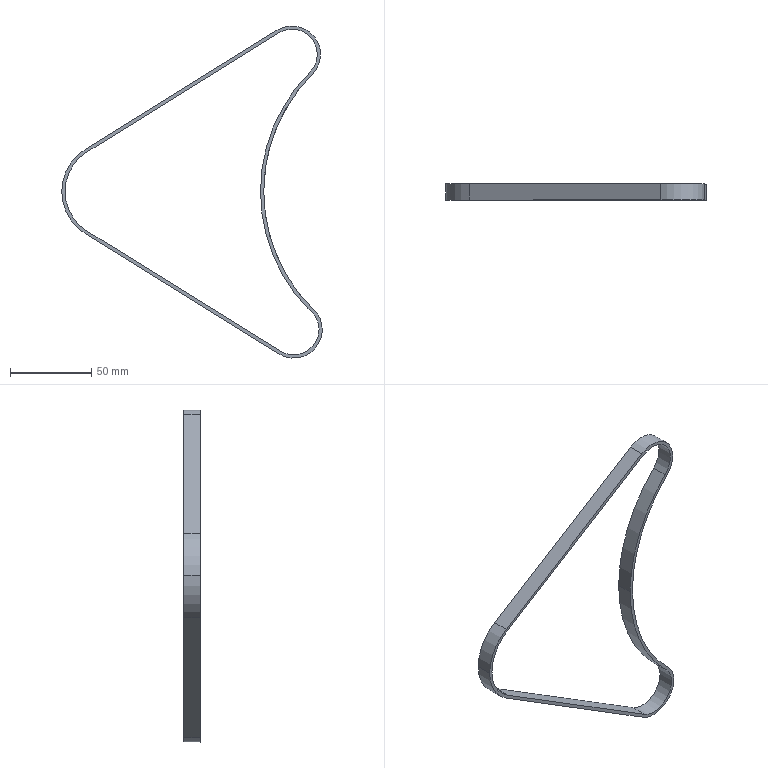Component | SolidWorks | Belt2-1 | 1 solid | 18 faces | box 159.92 x 10 x 203.95 mm | volume 11922 mm3 | cylinder 12 | plane 6 | commonest cylinder face diameters 207 x2 57 x2 203 x2 61 x2 31 x2 35 x2
STEP:
#1=COLOUR_RGB('',0.7922,0.8196,0.9333);
#2=FILL_AREA_STYLE_COLOUR('',#1);
#3=FILL_AREA_STYLE('',(#2));
#4=SURFACE_STYLE_FILL_AREA(#3);
#5=SURFACE_SIDE_STYLE('',(#4));
#6=SURFACE_STYLE_USAGE(.BOTH.,#5);
#7=PRESENTATION_STYLE_ASSIGNMENT((#6));
#8=CARTESIAN_POINT('',(0.02532,-2.067,3.386));
#9=VERTEX_POINT('',#8);
#10=CARTESIAN_POINT('',(-1.122,-2.067,6.22));
#11=VERTEX_POINT('',#10);
#12=CARTESIAN_POINT('',(2.953,-2.067,6.22));
#13=DIRECTION('',(0.,1.,0.));
#14=DIRECTION('',(1.,-0.,0.));
#15=AXIS2_PLACEMENT_3D('',#12,#13,#14);
#16=CIRCLE('',#15,4.075);
#17=EDGE_CURVE('',#9,#11,#16,.T.);
#18=ORIENTED_EDGE('',*,*,#17,.T.);
#19=CARTESIAN_POINT('',(-1.122,-1.673,6.22));
#20=VERTEX_POINT('',#19);
#21=CARTESIAN_POINT('',(-1.122,-2.067,6.22));
#22=DIRECTION('',(0.,1.,0.));
#23=VECTOR('',#22,39.37);
#24=LINE('',#21,#23);
#25=EDGE_CURVE('',#11,#20,#24,.T.);
#26=ORIENTED_EDGE('',*,*,#25,.T.);
#27=CARTESIAN_POINT('',(0.02532,-1.673,3.386));
#28=VERTEX_POINT('',#27);
#29=CARTESIAN_POINT('',(2.953,-1.673,6.22));
#30=DIRECTION('',(0.,1.,0.));
#31=DIRECTION('',(1.,-0.,0.));
#32=AXIS2_PLACEMENT_3D('',#29,#30,#31);
#33=CIRCLE('',#32,4.075);
#34=EDGE_CURVE('',#28,#20,#33,.T.);
#35=ORIENTED_EDGE('',*,*,#34,.F.);
#36=CARTESIAN_POINT('',(0.02532,-2.067,3.386));
#37=DIRECTION('',(0.,1.,0.));
#38=VECTOR('',#37,39.37);
#39=LINE('',#36,#38);
#40=EDGE_CURVE('',#9,#28,#39,.T.);
#41=ORIENTED_EDGE('',*,*,#40,.F.);
#42=EDGE_LOOP('',(#18,#26,#35,#41));
#43=FACE_OUTER_BOUND('',#42,.T.);
#44=CARTESIAN_POINT('',(2.953,-2.067,6.22));
#45=DIRECTION('',(0.,1.,0.));
#46=DIRECTION('',(-1.,0.,-0.));
#47=AXIS2_PLACEMENT_3D('',#44,#45,#46);
#48=CYLINDRICAL_SURFACE('',#47,4.075);
#49=ADVANCED_FACE('',(#43),#48,.T.);
#50=CARTESIAN_POINT('',(-5.316,-2.067,7.174));
#51=VERTEX_POINT('',#50);
#52=CARTESIAN_POINT('',(-5.846,-2.067,6.22));
#53=VERTEX_POINT('',#52);
#54=CARTESIAN_POINT('',(-4.724,-2.067,6.22));
#55=DIRECTION('',(-0.,-1.,-0.));
#56=DIRECTION('',(1.,-0.,0.));
#57=AXIS2_PLACEMENT_3D('',#54,#55,#56);
#58=CIRCLE('',#57,1.122);
#59=EDGE_CURVE('',#51,#53,#58,.T.);
#60=ORIENTED_EDGE('',*,*,#59,.T.);
#61=CARTESIAN_POINT('',(-5.846,-1.673,6.22));
#62=VERTEX_POINT('',#61);
#63=CARTESIAN_POINT('',(-5.846,-2.067,6.22));
#64=DIRECTION('',(0.,1.,0.));
#65=VECTOR('',#64,39.37);
#66=LINE('',#63,#65);
#67=EDGE_CURVE('',#53,#62,#66,.T.);
#68=ORIENTED_EDGE('',*,*,#67,.T.);
#69=CARTESIAN_POINT('',(-5.316,-1.673,7.174));
#70=VERTEX_POINT('',#69);
#71=CARTESIAN_POINT('',(-4.724,-1.673,6.22));
#72=DIRECTION('',(-0.,-1.,-0.));
#73=DIRECTION('',(1.,-0.,0.));
#74=AXIS2_PLACEMENT_3D('',#71,#72,#73);
#75=CIRCLE('',#74,1.122);
#76=EDGE_CURVE('',#70,#62,#75,.T.);
#77=ORIENTED_EDGE('',*,*,#76,.F.);
#78=CARTESIAN_POINT('',(-5.316,-2.067,7.174));
#79=DIRECTION('',(0.,1.,0.));
#80=VECTOR('',#79,39.37);
#81=LINE('',#78,#80);
#82=EDGE_CURVE('',#51,#70,#81,.T.);
#83=ORIENTED_EDGE('',*,*,#82,.F.);
#84=EDGE_LOOP('',(#60,#68,#77,#83));
#85=FACE_OUTER_BOUND('',#84,.T.);
#86=CARTESIAN_POINT('',(-4.724,-2.067,6.22));
#87=DIRECTION('',(0.,1.,0.));
#88=DIRECTION('',(-1.,0.,-0.));
#89=AXIS2_PLACEMENT_3D('',#86,#87,#88);
#90=CYLINDRICAL_SURFACE('',#89,1.122);
#91=ADVANCED_FACE('',(#85),#90,.F.);
#92=CARTESIAN_POINT('',(-1.043,-2.067,6.22));
#93=VERTEX_POINT('',#92);
#94=CARTESIAN_POINT('',(0.1271,-2.067,9.046));
#95=VERTEX_POINT('',#94);
#96=CARTESIAN_POINT('',(2.953,-2.067,6.22));
#97=DIRECTION('',(0.,1.,0.));
#98=DIRECTION('',(1.,-0.,0.));
#99=AXIS2_PLACEMENT_3D('',#96,#97,#98);
#100=CIRCLE('',#99,3.996);
#101=EDGE_CURVE('',#93,#95,#100,.T.);
#102=ORIENTED_EDGE('',*,*,#101,.F.);
#103=CARTESIAN_POINT('',(-1.043,-1.673,6.22));
#104=VERTEX_POINT('',#103);
#105=CARTESIAN_POINT('',(-1.043,-2.067,6.22));
#106=DIRECTION('',(0.,1.,0.));
#107=VECTOR('',#106,39.37);
#108=LINE('',#105,#107);
#109=EDGE_CURVE('',#93,#104,#108,.T.);
#110=ORIENTED_EDGE('',*,*,#109,.T.);
#111=CARTESIAN_POINT('',(0.1271,-1.673,9.046));
#112=VERTEX_POINT('',#111);
#113=CARTESIAN_POINT('',(-1.043,-1.673,6.22));
#114=CARTESIAN_POINT('',(-1.043,-1.673,6.482));
#115=CARTESIAN_POINT('',(-1.018,-1.673,6.744));
#116=CARTESIAN_POINT('',(-0.9155,-1.673,7.257));
#117=CARTESIAN_POINT('',(-0.8392,-1.673,7.508));
#118=CARTESIAN_POINT('',(-0.639,-1.673,7.991));
#119=CARTESIAN_POINT('',(-0.5152,-1.673,8.223));
#120=CARTESIAN_POINT('',(-0.2245,-1.673,8.658));
#121=CARTESIAN_POINT('',(-0.05783,-1.673,8.861));
#122=CARTESIAN_POINT('',(0.1271,-1.673,9.046));
#123=B_SPLINE_CURVE_WITH_KNOTS('',3,(#113,#114,#115,#116,#117,#118,#119,#120,#121,#122),.UNSPECIFIED.,.F.,.F.,(4,2,2,2,4),(0.4942,0.6206,0.7471,0.8735,1.),.UNSPECIFIED.);
#124=EDGE_CURVE('',#104,#112,#123,.T.);
#125=ORIENTED_EDGE('',*,*,#124,.T.);
#126=CARTESIAN_POINT('',(0.1271,-2.067,9.046));
#127=DIRECTION('',(0.,1.,0.));
#128=VECTOR('',#127,39.37);
#129=LINE('',#126,#128);
#130=EDGE_CURVE('',#95,#112,#129,.T.);
#131=ORIENTED_EDGE('',*,*,#130,.F.);
#132=EDGE_LOOP('',(#102,#110,#125,#131));
#133=FACE_OUTER_BOUND('',#132,.T.);
#134=CARTESIAN_POINT('',(2.953,-2.067,6.22));
#135=DIRECTION('',(0.,1.,0.));
#136=DIRECTION('',(-1.,0.,-0.));
#137=AXIS2_PLACEMENT_3D('',#134,#135,#136);
#138=CYLINDRICAL_SURFACE('',#137,3.996);
#139=ADVANCED_FACE('',(#133),#138,.F.);
#140=CARTESIAN_POINT('',(-5.925,-2.067,6.22));
#141=VERTEX_POINT('',#140);
#142=CARTESIAN_POINT('',(-5.358,-2.067,5.2));
#143=VERTEX_POINT('',#142);
#144=CARTESIAN_POINT('',(-4.724,-2.067,6.22));
#145=DIRECTION('',(-0.,-1.,-0.));
#146=DIRECTION('',(1.,-0.,0.));
#147=AXIS2_PLACEMENT_3D('',#144,#145,#146);
#148=CIRCLE('',#147,1.201);
#149=EDGE_CURVE('',#141,#143,#148,.T.);
#150=ORIENTED_EDGE('',*,*,#149,.F.);
#151=CARTESIAN_POINT('',(-5.925,-1.673,6.22));
#152=VERTEX_POINT('',#151);
#153=CARTESIAN_POINT('',(-5.925,-2.067,6.22));
#154=DIRECTION('',(0.,1.,0.));
#155=VECTOR('',#154,39.37);
#156=LINE('',#153,#155);
#157=EDGE_CURVE('',#141,#152,#156,.T.);
#158=ORIENTED_EDGE('',*,*,#157,.T.);
#159=CARTESIAN_POINT('',(-5.358,-1.673,5.2));
#160=VERTEX_POINT('',#159);
#161=CARTESIAN_POINT('',(-4.724,-1.673,6.22));
#162=DIRECTION('',(-0.,-1.,-0.));
#163=DIRECTION('',(1.,-0.,0.));
#164=AXIS2_PLACEMENT_3D('',#161,#162,#163);
#165=CIRCLE('',#164,1.201);
#166=EDGE_CURVE('',#152,#160,#165,.T.);
#167=ORIENTED_EDGE('',*,*,#166,.T.);
#168=CARTESIAN_POINT('',(-5.358,-2.067,5.2));
#169=DIRECTION('',(0.,1.,0.));
#170=VECTOR('',#169,39.37);
#171=LINE('',#168,#170);
#172=EDGE_CURVE('',#143,#160,#171,.T.);
#173=ORIENTED_EDGE('',*,*,#172,.F.);
#174=EDGE_LOOP('',(#150,#158,#167,#173));
#175=FACE_OUTER_BOUND('',#174,.T.);
#176=CARTESIAN_POINT('',(-4.724,-2.067,6.22));
#177=DIRECTION('',(0.,1.,0.));
#178=DIRECTION('',(-1.,0.,-0.));
#179=AXIS2_PLACEMENT_3D('',#176,#177,#178);
#180=CYLINDRICAL_SURFACE('',#179,1.201);
#181=ADVANCED_FACE('',(#175),#180,.T.);
#182=ORIENTED_EDGE('',*,*,#76,.T.);
#183=CARTESIAN_POINT('',(-5.316,-1.673,5.267));
#184=VERTEX_POINT('',#183);
#185=CARTESIAN_POINT('',(-4.724,-1.673,6.22));
#186=DIRECTION('',(-0.,-1.,-0.));
#187=DIRECTION('',(1.,-0.,0.));
#188=AXIS2_PLACEMENT_3D('',#185,#186,#187);
#189=CIRCLE('',#188,1.122);
#190=EDGE_CURVE('',#62,#184,#189,.T.);
#191=ORIENTED_EDGE('',*,*,#190,.T.);
#192=CARTESIAN_POINT('',(-0.6401,-1.673,2.363));
#193=VERTEX_POINT('',#192);
#194=CARTESIAN_POINT('',(-5.316,-1.673,5.267));
#195=DIRECTION('',(0.8495,0.,-0.5276));
#196=VECTOR('',#195,39.37);
#197=LINE('',#194,#196);
#198=EDGE_CURVE('',#184,#193,#197,.T.);
#199=ORIENTED_EDGE('',*,*,#198,.T.);
#200=CARTESIAN_POINT('',(-0.3181,-1.673,2.882));
#201=DIRECTION('',(-0.,-1.,-0.));
#202=DIRECTION('',(1.,-0.,0.));
#203=AXIS2_PLACEMENT_3D('',#200,#201,#202);
#204=CIRCLE('',#203,0.6102);
#205=EDGE_CURVE('',#193,#28,#204,.T.);
#206=ORIENTED_EDGE('',*,*,#205,.T.);
#207=ORIENTED_EDGE('',*,*,#34,.T.);
#208=CARTESIAN_POINT('',(0.07143,-1.673,9.102));
#209=VERTEX_POINT('',#208);
#210=CARTESIAN_POINT('',(2.953,-1.673,6.22));
#211=DIRECTION('',(0.,1.,0.));
#212=DIRECTION('',(1.,-0.,0.));
#213=AXIS2_PLACEMENT_3D('',#210,#211,#212);
#214=CIRCLE('',#213,4.075);
#215=EDGE_CURVE('',#20,#209,#214,.T.);
#216=ORIENTED_EDGE('',*,*,#215,.T.);
#217=CARTESIAN_POINT('',(-0.682,-1.673,10.052));
#218=VERTEX_POINT('',#217);
#219=CARTESIAN_POINT('',(-0.3601,-1.673,9.533));
#220=DIRECTION('',(-0.,-1.,-0.));
#221=DIRECTION('',(1.,-0.,0.));
#222=AXIS2_PLACEMENT_3D('',#219,#220,#221);
#223=CIRCLE('',#222,0.6102);
#224=EDGE_CURVE('',#209,#218,#223,.T.);
#225=ORIENTED_EDGE('',*,*,#224,.T.);
#226=CARTESIAN_POINT('',(-5.316,-1.673,7.174));
#227=DIRECTION('',(-0.8495,0.,-0.5276));
#228=VECTOR('',#227,39.37);
#229=LINE('',#226,#228);
#230=EDGE_CURVE('',#218,#70,#229,.T.);
#231=ORIENTED_EDGE('',*,*,#230,.T.);
#232=EDGE_LOOP('',(#182,#191,#199,#206,#207,#216,#225,#231));
#233=FACE_BOUND('',#232,.T.);
#234=CARTESIAN_POINT('',(0.2385,-1.673,3.288));
#235=VERTEX_POINT('',#234);
#236=CARTESIAN_POINT('',(0.07649,-1.673,3.446));
#237=VERTEX_POINT('',#236);
#238=CARTESIAN_POINT('',(0.2385,-1.673,3.288));
#239=CARTESIAN_POINT('',(0.2107,-1.673,3.313));
#240=CARTESIAN_POINT('',(0.156,-1.673,3.365));
#241=CARTESIAN_POINT('',(0.1027,-1.673,3.419));
#242=CARTESIAN_POINT('',(0.07649,-1.673,3.446));
#243=B_SPLINE_CURVE_WITH_KNOTS('',3,(#238,#239,#240,#241,#242),.UNSPECIFIED.,.F.,.F.,(4,1,4),(0.8688,0.8734,0.8779),.UNSPECIFIED.);
#244=EDGE_CURVE('',#235,#237,#243,.T.);
#245=ORIENTED_EDGE('',*,*,#244,.F.);
#246=CARTESIAN_POINT('',(-0.6816,-1.673,2.296));
#247=VERTEX_POINT('',#246);
#248=CARTESIAN_POINT('',(-0.3181,-1.673,2.882));
#249=DIRECTION('',(-0.,-1.,-0.));
#250=DIRECTION('',(-1.,0.,-0.));
#251=AXIS2_PLACEMENT_3D('',#248,#249,#250);
#252=CIRCLE('',#251,0.689);
#253=EDGE_CURVE('',#247,#235,#252,.T.);
#254=ORIENTED_EDGE('',*,*,#253,.F.);
#255=CARTESIAN_POINT('',(-5.358,-1.673,5.2));
#256=DIRECTION('',(0.8495,0.,-0.5276));
#257=VECTOR('',#256,39.37);
#258=LINE('',#255,#257);
#259=EDGE_CURVE('',#160,#247,#258,.T.);
#260=ORIENTED_EDGE('',*,*,#259,.F.);
#261=ORIENTED_EDGE('',*,*,#166,.F.);
#262=CARTESIAN_POINT('',(-5.358,-1.673,7.241));
#263=VERTEX_POINT('',#262);
#264=CARTESIAN_POINT('',(-4.724,-1.673,6.22));
#265=DIRECTION('',(-0.,-1.,-0.));
#266=DIRECTION('',(1.,-0.,0.));
#267=AXIS2_PLACEMENT_3D('',#264,#265,#266);
#268=CIRCLE('',#267,1.201);
#269=EDGE_CURVE('',#263,#152,#268,.T.);
#270=ORIENTED_EDGE('',*,*,#269,.F.);
#271=CARTESIAN_POINT('',(-0.7235,-1.673,10.119));
#272=VERTEX_POINT('',#271);
#273=CARTESIAN_POINT('',(-5.358,-1.673,7.241));
#274=DIRECTION('',(-0.8495,0.,-0.5276));
#275=VECTOR('',#274,39.37);
#276=LINE('',#273,#275);
#277=EDGE_CURVE('',#272,#263,#276,.T.);
#278=ORIENTED_EDGE('',*,*,#277,.F.);
#279=CARTESIAN_POINT('',(-0.3601,-1.673,9.533));
#280=DIRECTION('',(-0.,-1.,-0.));
#281=DIRECTION('',(1.,-0.,0.));
#282=AXIS2_PLACEMENT_3D('',#279,#280,#281);
#283=CIRCLE('',#282,0.689);
#284=EDGE_CURVE('',#112,#272,#283,.T.);
#285=ORIENTED_EDGE('',*,*,#284,.F.);
#286=ORIENTED_EDGE('',*,*,#124,.F.);
#287=CARTESIAN_POINT('',(0.07649,-1.673,3.446));
#288=CARTESIAN_POINT('',(-0.1009,-1.673,3.63));
#289=CARTESIAN_POINT('',(-0.2606,-1.673,3.831));
#290=CARTESIAN_POINT('',(-0.5387,-1.673,4.26));
#291=CARTESIAN_POINT('',(-0.6572,-1.673,4.488));
#292=CARTESIAN_POINT('',(-0.8484,-1.673,4.962));
#293=CARTESIAN_POINT('',(-0.9213,-1.673,5.208));
#294=CARTESIAN_POINT('',(-1.019,-1.673,5.709));
#295=CARTESIAN_POINT('',(-1.043,-1.673,5.965));
#296=CARTESIAN_POINT('',(-1.043,-1.673,6.22));
#297=B_SPLINE_CURVE_WITH_KNOTS('',3,(#287,#288,#289,#290,#291,#292,#293,#294,#295,#296),.UNSPECIFIED.,.F.,.F.,(4,2,2,2,4),(0.,0.1235,0.2471,0.3706,0.4942),.UNSPECIFIED.);
#298=EDGE_CURVE('',#237,#104,#297,.T.);
#299=ORIENTED_EDGE('',*,*,#298,.F.);
#300=EDGE_LOOP('',(#245,#254,#260,#261,#270,#278,#285,#286,#299));
#301=FACE_OUTER_BOUND('',#300,.T.);
#302=CARTESIAN_POINT('',(-4.724,-1.673,6.22));
#303=DIRECTION('',(-0.,-1.,-0.));
#304=DIRECTION('',(-0.,-0.,1.));
#305=AXIS2_PLACEMENT_3D('',#302,#303,#304);
#306=PLANE('',#305);
#307=ADVANCED_FACE('',(#233,#301),#306,.F.);
#308=CARTESIAN_POINT('',(-5.316,-2.067,5.267));
#309=VERTEX_POINT('',#308);
#310=CARTESIAN_POINT('',(-0.6401,-2.067,2.363));
#311=VERTEX_POINT('',#310);
#312=CARTESIAN_POINT('',(-5.316,-2.067,5.267));
#313=DIRECTION('',(0.8495,0.,-0.5276));
#314=VECTOR('',#313,39.37);
#315=LINE('',#312,#314);
#316=EDGE_CURVE('',#309,#311,#315,.T.);
#317=ORIENTED_EDGE('',*,*,#316,.F.);
#318=CARTESIAN_POINT('',(-4.724,-2.067,6.22));
#319=DIRECTION('',(-0.,-1.,-0.));
#320=DIRECTION('',(1.,-0.,0.));
#321=AXIS2_PLACEMENT_3D('',#318,#319,#320);
#322=CIRCLE('',#321,1.122);
#323=EDGE_CURVE('',#53,#309,#322,.T.);
#324=ORIENTED_EDGE('',*,*,#323,.F.);
#325=ORIENTED_EDGE('',*,*,#59,.F.);
#326=CARTESIAN_POINT('',(-0.682,-2.067,10.052));
#327=VERTEX_POINT('',#326);
#328=CARTESIAN_POINT('',(-5.316,-2.067,7.174));
#329=DIRECTION('',(-0.8495,0.,-0.5276));
#330=VECTOR('',#329,39.37);
#331=LINE('',#328,#330);
#332=EDGE_CURVE('',#327,#51,#331,.T.);
#333=ORIENTED_EDGE('',*,*,#332,.F.);
#334=CARTESIAN_POINT('',(0.07143,-2.067,9.102));
#335=VERTEX_POINT('',#334);
#336=CARTESIAN_POINT('',(-0.3601,-2.067,9.533));
#337=DIRECTION('',(-0.,-1.,-0.));
#338=DIRECTION('',(1.,-0.,0.));
#339=AXIS2_PLACEMENT_3D('',#336,#337,#338);
#340=CIRCLE('',#339,0.6102);
#341=EDGE_CURVE('',#335,#327,#340,.T.);
#342=ORIENTED_EDGE('',*,*,#341,.F.);
#343=CARTESIAN_POINT('',(2.953,-2.067,6.22));
#344=DIRECTION('',(0.,1.,0.));
#345=DIRECTION('',(1.,-0.,0.));
#346=AXIS2_PLACEMENT_3D('',#343,#344,#345);
#347=CIRCLE('',#346,4.075);
#348=EDGE_CURVE('',#11,#335,#347,.T.);
#349=ORIENTED_EDGE('',*,*,#348,.F.);
#350=ORIENTED_EDGE('',*,*,#17,.F.);
#351=CARTESIAN_POINT('',(-0.3181,-2.067,2.882));
#352=DIRECTION('',(-0.,-1.,-0.));
#353=DIRECTION('',(1.,-0.,0.));
#354=AXIS2_PLACEMENT_3D('',#351,#352,#353);
#355=CIRCLE('',#354,0.6102);
#356=EDGE_CURVE('',#311,#9,#355,.T.);
#357=ORIENTED_EDGE('',*,*,#356,.F.);
#358=EDGE_LOOP('',(#317,#324,#325,#333,#342,#349,#350,#357));
#359=FACE_BOUND('',#358,.T.);
#360=CARTESIAN_POINT('',(-0.6816,-2.067,2.296));
#361=VERTEX_POINT('',#360);
#362=CARTESIAN_POINT('',(0.2384,-2.067,3.288));
#363=VERTEX_POINT('',#362);
#364=CARTESIAN_POINT('',(-0.3181,-2.067,2.882));
#365=DIRECTION('',(-0.,-1.,-0.));
#366=DIRECTION('',(1.,-0.,0.));
#367=AXIS2_PLACEMENT_3D('',#364,#365,#366);
#368=CIRCLE('',#367,0.689);
#369=EDGE_CURVE('',#361,#363,#368,.T.);
#370=ORIENTED_EDGE('',*,*,#369,.T.);
#371=CARTESIAN_POINT('',(2.953,-2.067,6.22));
#372=DIRECTION('',(0.,1.,0.));
#373=DIRECTION('',(1.,-0.,0.));
#374=AXIS2_PLACEMENT_3D('',#371,#372,#373);
#375=CIRCLE('',#374,3.996);
#376=EDGE_CURVE('',#363,#93,#375,.T.);
#377=ORIENTED_EDGE('',*,*,#376,.T.);
#378=ORIENTED_EDGE('',*,*,#101,.T.);
#379=CARTESIAN_POINT('',(-0.7235,-2.067,10.119));
#380=VERTEX_POINT('',#379);
#381=CARTESIAN_POINT('',(-0.3601,-2.067,9.533));
#382=DIRECTION('',(-0.,-1.,-0.));
#383=DIRECTION('',(1.,-0.,0.));
#384=AXIS2_PLACEMENT_3D('',#381,#382,#383);
#385=CIRCLE('',#384,0.689);
#386=EDGE_CURVE('',#95,#380,#385,.T.);
#387=ORIENTED_EDGE('',*,*,#386,.T.);
#388=CARTESIAN_POINT('',(-5.358,-2.067,7.241));
#389=VERTEX_POINT('',#388);
#390=CARTESIAN_POINT('',(-5.358,-2.067,7.241));
#391=DIRECTION('',(-0.8495,0.,-0.5276));
#392=VECTOR('',#391,39.37);
#393=LINE('',#390,#392);
#394=EDGE_CURVE('',#380,#389,#393,.T.);
#395=ORIENTED_EDGE('',*,*,#394,.T.);
#396=CARTESIAN_POINT('',(-4.724,-2.067,6.22));
#397=DIRECTION('',(-0.,-1.,-0.));
#398=DIRECTION('',(1.,-0.,0.));
#399=AXIS2_PLACEMENT_3D('',#396,#397,#398);
#400=CIRCLE('',#399,1.201);
#401=EDGE_CURVE('',#389,#141,#400,.T.);
#402=ORIENTED_EDGE('',*,*,#401,.T.);
#403=ORIENTED_EDGE('',*,*,#149,.T.);
#404=CARTESIAN_POINT('',(-5.358,-2.067,5.2));
#405=DIRECTION('',(0.8495,0.,-0.5276));
#406=VECTOR('',#405,39.37);
#407=LINE('',#404,#406);
#408=EDGE_CURVE('',#143,#361,#407,.T.);
#409=ORIENTED_EDGE('',*,*,#408,.T.);
#410=EDGE_LOOP('',(#370,#377,#378,#387,#395,#402,#403,#409));
#411=FACE_OUTER_BOUND('',#410,.T.);
#412=CARTESIAN_POINT('',(-4.724,-2.067,6.22));
#413=DIRECTION('',(-0.,-1.,-0.));
#414=DIRECTION('',(-0.,-0.,1.));
#415=AXIS2_PLACEMENT_3D('',#412,#413,#414);
#416=PLANE('',#415);
#417=ADVANCED_FACE('',(#359,#411),#416,.T.);
#418=ORIENTED_EDGE('',*,*,#230,.F.);
#419=CARTESIAN_POINT('',(-0.682,-2.067,10.052));
#420=DIRECTION('',(0.,1.,0.));
#421=VECTOR('',#420,39.37);
#422=LINE('',#419,#421);
#423=EDGE_CURVE('',#327,#218,#422,.T.);
#424=ORIENTED_EDGE('',*,*,#423,.F.);
#425=ORIENTED_EDGE('',*,*,#332,.T.);
#426=ORIENTED_EDGE('',*,*,#82,.T.);
#427=EDGE_LOOP('',(#418,#424,#425,#426));
#428=FACE_OUTER_BOUND('',#427,.T.);
#429=CARTESIAN_POINT('',(-5.316,-2.067,7.174));
#430=DIRECTION('',(0.5276,0.,-0.8495));
#431=DIRECTION('',(0.8495,-0.,0.5276));
#432=AXIS2_PLACEMENT_3D('',#429,#430,#431);
#433=PLANE('',#432);
#434=ADVANCED_FACE('',(#428),#433,.T.);
#435=ORIENTED_EDGE('',*,*,#224,.F.);
#436=CARTESIAN_POINT('',(0.07143,-2.067,9.102));
#437=DIRECTION('',(0.,1.,0.));
#438=VECTOR('',#437,39.37);
#439=LINE('',#436,#438);
#440=EDGE_CURVE('',#335,#209,#439,.T.);
#441=ORIENTED_EDGE('',*,*,#440,.F.);
#442=ORIENTED_EDGE('',*,*,#341,.T.);
#443=ORIENTED_EDGE('',*,*,#423,.T.);
#444=EDGE_LOOP('',(#435,#441,#442,#443));
#445=FACE_OUTER_BOUND('',#444,.T.);
#446=CARTESIAN_POINT('',(-0.3601,-2.067,9.533));
#447=DIRECTION('',(0.,1.,0.));
#448=DIRECTION('',(-1.,0.,-0.));
#449=AXIS2_PLACEMENT_3D('',#446,#447,#448);
#450=CYLINDRICAL_SURFACE('',#449,0.6102);
#451=ADVANCED_FACE('',(#445),#450,.F.);
#452=ORIENTED_EDGE('',*,*,#205,.F.);
#453=CARTESIAN_POINT('',(-0.6401,-2.067,2.363));
#454=DIRECTION('',(0.,1.,0.));
#455=VECTOR('',#454,39.37);
#456=LINE('',#453,#455);
#457=EDGE_CURVE('',#311,#193,#456,.T.);
#458=ORIENTED_EDGE('',*,*,#457,.F.);
#459=ORIENTED_EDGE('',*,*,#356,.T.);
#460=ORIENTED_EDGE('',*,*,#40,.T.);
#461=EDGE_LOOP('',(#452,#458,#459,#460));
#462=FACE_OUTER_BOUND('',#461,.T.);
#463=CARTESIAN_POINT('',(-0.3181,-2.067,2.882));
#464=DIRECTION('',(0.,1.,0.));
#465=DIRECTION('',(-1.,0.,-0.));
#466=AXIS2_PLACEMENT_3D('',#463,#464,#465);
#467=CYLINDRICAL_SURFACE('',#466,0.6102);
#468=ADVANCED_FACE('',(#462),#467,.F.);
#469=ORIENTED_EDGE('',*,*,#198,.F.);
#470=CARTESIAN_POINT('',(-5.316,-2.067,5.267));
#471=DIRECTION('',(0.,1.,0.));
#472=VECTOR('',#471,39.37);
#473=LINE('',#470,#472);
#474=EDGE_CURVE('',#309,#184,#473,.T.);
#475=ORIENTED_EDGE('',*,*,#474,.F.);
#476=ORIENTED_EDGE('',*,*,#316,.T.);
#477=ORIENTED_EDGE('',*,*,#457,.T.);
#478=EDGE_LOOP('',(#469,#475,#476,#477));
#479=FACE_OUTER_BOUND('',#478,.T.);
#480=CARTESIAN_POINT('',(-5.316,-2.067,5.267));
#481=DIRECTION('',(0.5276,-0.,0.8495));
#482=DIRECTION('',(0.,1.,0.));
#483=AXIS2_PLACEMENT_3D('',#480,#481,#482);
#484=PLANE('',#483);
#485=ADVANCED_FACE('',(#479),#484,.T.);
#486=ORIENTED_EDGE('',*,*,#277,.T.);
#487=CARTESIAN_POINT('',(-5.358,-2.067,7.241));
#488=DIRECTION('',(0.,1.,0.));
#489=VECTOR('',#488,39.37);
#490=LINE('',#487,#489);
#491=EDGE_CURVE('',#389,#263,#490,.T.);
#492=ORIENTED_EDGE('',*,*,#491,.F.);
#493=ORIENTED_EDGE('',*,*,#394,.F.);
#494=CARTESIAN_POINT('',(-0.7235,-2.067,10.119));
#495=DIRECTION('',(0.,1.,0.));
#496=VECTOR('',#495,39.37);
#497=LINE('',#494,#496);
#498=EDGE_CURVE('',#380,#272,#497,.T.);
#499=ORIENTED_EDGE('',*,*,#498,.T.);
#500=EDGE_LOOP('',(#486,#492,#493,#499));
#501=FACE_OUTER_BOUND('',#500,.T.);
#502=CARTESIAN_POINT('',(-5.358,-2.067,7.241));
#503=DIRECTION('',(0.5276,0.,-0.8495));
#504=DIRECTION('',(0.8495,-0.,0.5276));
#505=AXIS2_PLACEMENT_3D('',#502,#503,#504);
#506=PLANE('',#505);
#507=ADVANCED_FACE('',(#501),#506,.F.);
#508=ORIENTED_EDGE('',*,*,#284,.T.);
#509=ORIENTED_EDGE('',*,*,#498,.F.);
#510=ORIENTED_EDGE('',*,*,#386,.F.);
#511=ORIENTED_EDGE('',*,*,#130,.T.);
#512=EDGE_LOOP('',(#508,#509,#510,#511));
#513=FACE_OUTER_BOUND('',#512,.T.);
#514=CARTESIAN_POINT('',(-0.3601,-2.067,9.533));
#515=DIRECTION('',(0.,1.,0.));
#516=DIRECTION('',(-1.,0.,-0.));
#517=AXIS2_PLACEMENT_3D('',#514,#515,#516);
#518=CYLINDRICAL_SURFACE('',#517,0.689);
#519=ADVANCED_FACE('',(#513),#518,.T.);
#520=CARTESIAN_POINT('',(0.2384,-1.87,3.288));
#521=DIRECTION('',(0.,1.,0.));
#522=VECTOR('',#521,39.37);
#523=LINE('',#520,#522);
#524=EDGE_CURVE('',#363,#235,#523,.T.);
#525=ORIENTED_EDGE('',*,*,#524,.F.);
#526=ORIENTED_EDGE('',*,*,#369,.F.);
#527=CARTESIAN_POINT('',(-0.6816,-2.067,2.296));
#528=DIRECTION('',(0.,1.,0.));
#529=VECTOR('',#528,39.37);
#530=LINE('',#527,#529);
#531=EDGE_CURVE('',#361,#247,#530,.T.);
#532=ORIENTED_EDGE('',*,*,#531,.T.);
#533=ORIENTED_EDGE('',*,*,#253,.T.);
#534=EDGE_LOOP('',(#525,#526,#532,#533));
#535=FACE_OUTER_BOUND('',#534,.T.);
#536=CARTESIAN_POINT('',(-0.3181,-2.067,2.882));
#537=DIRECTION('',(0.,1.,0.));
#538=DIRECTION('',(-1.,0.,-0.));
#539=AXIS2_PLACEMENT_3D('',#536,#537,#538);
#540=CYLINDRICAL_SURFACE('',#539,0.689);
#541=ADVANCED_FACE('',(#535),#540,.T.);
#542=ORIENTED_EDGE('',*,*,#259,.T.);
#543=ORIENTED_EDGE('',*,*,#531,.F.);
#544=ORIENTED_EDGE('',*,*,#408,.F.);
#545=ORIENTED_EDGE('',*,*,#172,.T.);
#546=EDGE_LOOP('',(#542,#543,#544,#545));
#547=FACE_OUTER_BOUND('',#546,.T.);
#548=CARTESIAN_POINT('',(-5.358,-2.067,5.2));
#549=DIRECTION('',(0.5276,-0.,0.8495));
#550=DIRECTION('',(0.,1.,0.));
#551=AXIS2_PLACEMENT_3D('',#548,#549,#550);
#552=PLANE('',#551);
#553=ADVANCED_FACE('',(#547),#552,.F.);
#554=ORIENTED_EDGE('',*,*,#157,.F.);
#555=ORIENTED_EDGE('',*,*,#401,.F.);
#556=ORIENTED_EDGE('',*,*,#491,.T.);
#557=ORIENTED_EDGE('',*,*,#269,.T.);
#558=EDGE_LOOP('',(#554,#555,#556,#557));
#559=FACE_OUTER_BOUND('',#558,.T.);
#560=CARTESIAN_POINT('',(-4.724,-2.067,6.22));
#561=DIRECTION('',(0.,1.,0.));
#562=DIRECTION('',(-1.,0.,-0.));
#563=AXIS2_PLACEMENT_3D('',#560,#561,#562);
#564=CYLINDRICAL_SURFACE('',#563,1.201);
#565=ADVANCED_FACE('',(#559),#564,.T.);
#566=ORIENTED_EDGE('',*,*,#109,.F.);
#567=ORIENTED_EDGE('',*,*,#376,.F.);
#568=ORIENTED_EDGE('',*,*,#524,.T.);
#569=ORIENTED_EDGE('',*,*,#244,.T.);
#570=ORIENTED_EDGE('',*,*,#298,.T.);
#571=EDGE_LOOP('',(#566,#567,#568,#569,#570));
#572=FACE_OUTER_BOUND('',#571,.T.);
#573=CARTESIAN_POINT('',(2.953,-2.067,6.22));
#574=DIRECTION('',(0.,1.,0.));
#575=DIRECTION('',(-1.,0.,-0.));
#576=AXIS2_PLACEMENT_3D('',#573,#574,#575);
#577=CYLINDRICAL_SURFACE('',#576,3.996);
#578=ADVANCED_FACE('',(#572),#577,.F.);
#579=ORIENTED_EDGE('',*,*,#67,.F.);
#580=ORIENTED_EDGE('',*,*,#323,.T.);
#581=ORIENTED_EDGE('',*,*,#474,.T.);
#582=ORIENTED_EDGE('',*,*,#190,.F.);
#583=EDGE_LOOP('',(#579,#580,#581,#582));
#584=FACE_OUTER_BOUND('',#583,.T.);
#585=CARTESIAN_POINT('',(-4.724,-2.067,6.22));
#586=DIRECTION('',(0.,1.,0.));
#587=DIRECTION('',(-1.,0.,-0.));
#588=AXIS2_PLACEMENT_3D('',#585,#586,#587);
#589=CYLINDRICAL_SURFACE('',#588,1.122);
#590=ADVANCED_FACE('',(#584),#589,.F.);
#591=ORIENTED_EDGE('',*,*,#25,.F.);
#592=ORIENTED_EDGE('',*,*,#348,.T.);
#593=ORIENTED_EDGE('',*,*,#440,.T.);
#594=ORIENTED_EDGE('',*,*,#215,.F.);
#595=EDGE_LOOP('',(#591,#592,#593,#594));
#596=FACE_OUTER_BOUND('',#595,.T.);
#597=CARTESIAN_POINT('',(2.953,-2.067,6.22));
#598=DIRECTION('',(0.,1.,0.));
#599=DIRECTION('',(-1.,0.,-0.));
#600=AXIS2_PLACEMENT_3D('',#597,#598,#599);
#601=CYLINDRICAL_SURFACE('',#600,4.075);
#602=ADVANCED_FACE('',(#596),#601,.T.);
#603=CLOSED_SHELL('',(#49,#91,#139,#181,#307,#417,#434,#451,#468,#485,#507,#519,#541,#553,#565,#578,#590,#602));
#604=MANIFOLD_SOLID_BREP('',#603);
#605=STYLED_ITEM('',(#7),#604);
#606=PRESENTATION_LAYER_ASSIGNMENT('','',(#605));
#607=(LENGTH_UNIT()NAMED_UNIT(*)SI_UNIT($,.METRE.));
#608=LENGTH_MEASURE_WITH_UNIT(LENGTH_MEASURE(0.0254),#607);
#609=DIMENSIONAL_EXPONENTS(1.,0.,0.,0.,0.,0.,0.);
#610=(CONVERSION_BASED_UNIT('',#608)LENGTH_UNIT()NAMED_UNIT(#609));
#611=UNCERTAINTY_MEASURE_WITH_UNIT(LENGTH_MEASURE(0.00001),#610,'','');
#612=(NAMED_UNIT(*)PLANE_ANGLE_UNIT()SI_UNIT($,.RADIAN.));
#613=(NAMED_UNIT(*)SI_UNIT($,.STERADIAN.)SOLID_ANGLE_UNIT());
#614=(GEOMETRIC_REPRESENTATION_CONTEXT(3)GLOBAL_UNCERTAINTY_ASSIGNED_CONTEXT((#611))GLOBAL_UNIT_ASSIGNED_CONTEXT((#610,#612,#613))REPRESENTATION_CONTEXT('',''));
#615=MECHANICAL_DESIGN_GEOMETRIC_PRESENTATION_REPRESENTATION('',(#605),#614);
#616=CARTESIAN_POINT('',(0.,0.,0.));
#617=DIRECTION('',(0.,0.,1.));
#618=DIRECTION('',(1.,0.,0.));
#619=AXIS2_PLACEMENT_3D('',#616,#617,#618);
#620=(LENGTH_UNIT()NAMED_UNIT(*)SI_UNIT($,.METRE.));
#621=LENGTH_MEASURE_WITH_UNIT(LENGTH_MEASURE(0.0254),#620);
#622=DIMENSIONAL_EXPONENTS(1.,0.,0.,0.,0.,0.,0.);
#623=(CONVERSION_BASED_UNIT('',#621)LENGTH_UNIT()NAMED_UNIT(#622));
#624=UNCERTAINTY_MEASURE_WITH_UNIT(LENGTH_MEASURE(0.00001),#623,'','');
#625=(NAMED_UNIT(*)PLANE_ANGLE_UNIT()SI_UNIT($,.RADIAN.));
#626=(NAMED_UNIT(*)SI_UNIT($,.STERADIAN.)SOLID_ANGLE_UNIT());
#627=(GEOMETRIC_REPRESENTATION_CONTEXT(3)GLOBAL_UNCERTAINTY_ASSIGNED_CONTEXT((#624))GLOBAL_UNIT_ASSIGNED_CONTEXT((#623,#625,#626))REPRESENTATION_CONTEXT('',''));
#628=ADVANCED_BREP_SHAPE_REPRESENTATION('',(#604,#619),#627);